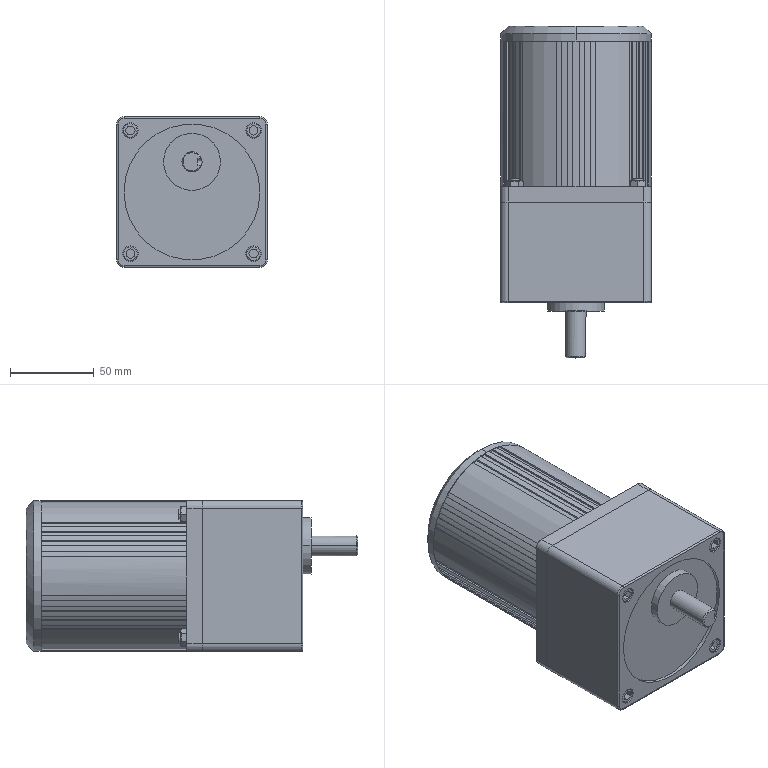Component | SolidWorks | IK-AC(40W)InductionMotor[5IK40A1-C]-1 | 3 solids | 335 faces | volume 1156933 mm3 | plane 188 | cylinder 96 | cone 39 | torus 12 | commonest cylinder face diameters 90 x27 88 x24 9 x16 6 x8 9.2 x8 1.8 x4 89.8 x2 34 x2